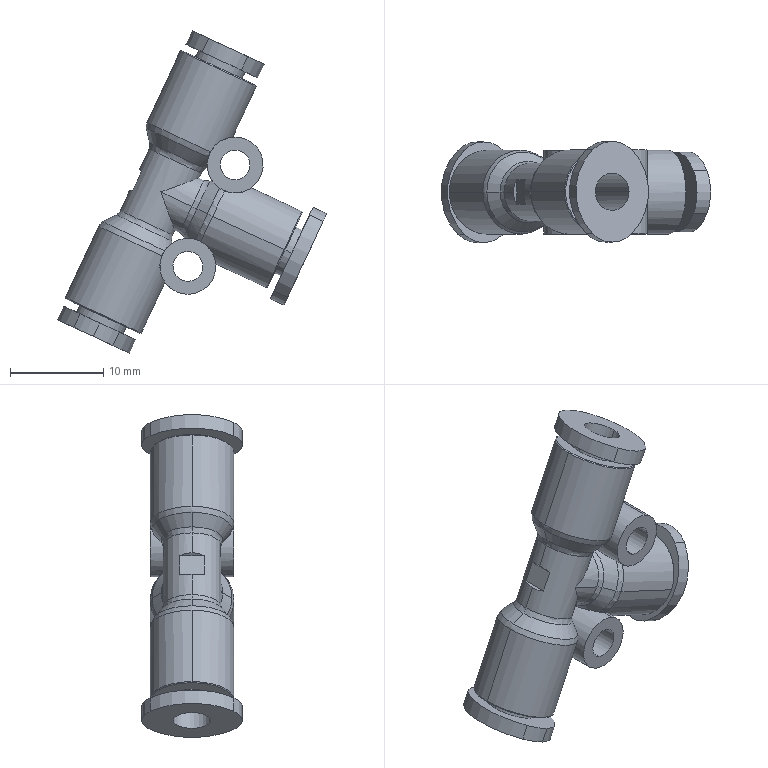Component | SolidWorks | T-Joint-1 | 1 solid | 92 faces | volume 2358 mm3 | cylinder 50 | plane 19 | cone 12 | spline 11 | commonest cylinder face diameters 6.862 x8 12.192 x7 9 x6 5.5 x6 4 x6 2 x5 6 x4 3.2 x4